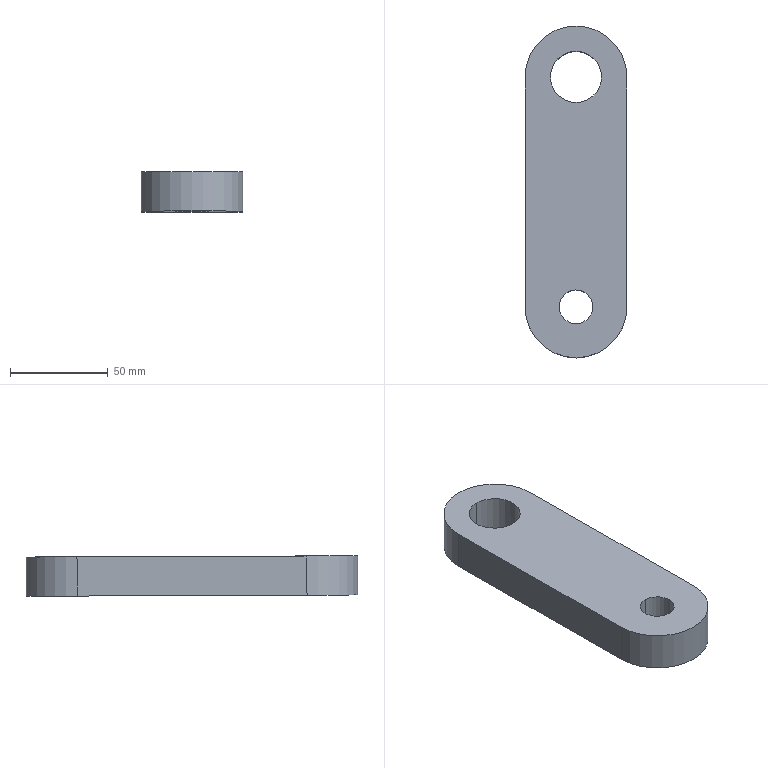Component | SolidWorks | RehabilitationChair-18-18-1 | 1 solid | 11 faces | box 52.03 x 169.45 x 20.64 mm | volume 149257 mm3 | cylinder 7 | plane 4 | commonest cylinder face diameters 52.026 x3 26.129 x2 17.187 x2
STEP:
#1=COLOUR_RGB('',0.7922,0.8196,0.9333);
#2=FILL_AREA_STYLE_COLOUR('',#1);
#3=FILL_AREA_STYLE('',(#2));
#4=SURFACE_STYLE_FILL_AREA(#3);
#5=SURFACE_SIDE_STYLE('',(#4));
#6=SURFACE_STYLE_USAGE(.BOTH.,#5);
#7=PRESENTATION_STYLE_ASSIGNMENT((#6));
#8=CARTESIAN_POINT('',(12.719,14.763,13.988));
#9=VERTEX_POINT('',#8);
#10=CARTESIAN_POINT('',(12.719,15.792,13.984));
#11=VERTEX_POINT('',#10);
#12=CARTESIAN_POINT('',(12.719,15.278,13.986));
#13=DIRECTION('',(-0.0003323,0.003798,1.));
#14=DIRECTION('',(0.,1.,-0.003798));
#15=AXIS2_PLACEMENT_3D('',#12,#13,#14);
#16=CIRCLE('',#15,0.5144);
#17=EDGE_CURVE('',#9,#11,#16,.T.);
#18=ORIENTED_EDGE('',*,*,#17,.T.);
#19=CARTESIAN_POINT('',(12.719,15.789,13.197));
#20=VERTEX_POINT('',#19);
#21=CARTESIAN_POINT('',(12.718,15.802,16.73));
#22=DIRECTION('',(0.0003323,-0.003798,-1.));
#23=VECTOR('',#22,39.37);
#24=LINE('',#21,#23);
#25=EDGE_CURVE('',#11,#20,#24,.T.);
#26=ORIENTED_EDGE('',*,*,#25,.T.);
#27=CARTESIAN_POINT('',(12.719,14.76,13.201));
#28=VERTEX_POINT('',#27);
#29=CARTESIAN_POINT('',(12.719,15.275,13.199));
#30=DIRECTION('',(-0.0003323,0.003798,1.));
#31=DIRECTION('',(0.,-1.,0.003798));
#32=AXIS2_PLACEMENT_3D('',#29,#30,#31);
#33=CIRCLE('',#32,0.5144);
#34=EDGE_CURVE('',#28,#20,#33,.T.);
#35=ORIENTED_EDGE('',*,*,#34,.F.);
#36=CARTESIAN_POINT('',(12.718,14.774,16.734));
#37=DIRECTION('',(0.0003323,-0.003798,-1.));
#38=VECTOR('',#37,39.37);
#39=LINE('',#36,#38);
#40=EDGE_CURVE('',#9,#28,#39,.T.);
#41=ORIENTED_EDGE('',*,*,#40,.F.);
#42=EDGE_LOOP('',(#18,#26,#35,#41));
#43=FACE_OUTER_BOUND('',#42,.T.);
#44=CARTESIAN_POINT('',(12.718,15.288,16.732));
#45=DIRECTION('',(0.0003323,-0.003798,-1.));
#46=DIRECTION('',(0.,-1.,0.003798));
#47=AXIS2_PLACEMENT_3D('',#44,#45,#46);
#48=CYLINDRICAL_SURFACE('',#47,0.5144);
#49=ADVANCED_FACE('',(#43),#48,.F.);
#50=CARTESIAN_POINT('',(12.719,10.996,14.002));
#51=VERTEX_POINT('',#50);
#52=CARTESIAN_POINT('',(12.719,10.319,14.005));
#53=VERTEX_POINT('',#52);
#54=CARTESIAN_POINT('',(12.719,10.658,14.004));
#55=DIRECTION('',(0.0003323,-0.003798,-1.));
#56=DIRECTION('',(0.,1.,-0.003798));
#57=AXIS2_PLACEMENT_3D('',#54,#55,#56);
#58=CIRCLE('',#57,0.3383);
#59=EDGE_CURVE('',#51,#53,#58,.T.);
#60=ORIENTED_EDGE('',*,*,#59,.F.);
#61=CARTESIAN_POINT('',(12.719,10.993,13.215));
#62=VERTEX_POINT('',#61);
#63=CARTESIAN_POINT('',(12.718,11.007,16.8));
#64=DIRECTION('',(0.0003323,-0.003798,-1.));
#65=VECTOR('',#64,39.37);
#66=LINE('',#63,#65);
#67=EDGE_CURVE('',#51,#62,#66,.T.);
#68=ORIENTED_EDGE('',*,*,#67,.T.);
#69=CARTESIAN_POINT('',(12.719,10.316,13.218));
#70=VERTEX_POINT('',#69);
#71=CARTESIAN_POINT('',(12.719,10.655,13.216));
#72=DIRECTION('',(-0.0003323,0.003798,1.));
#73=DIRECTION('',(0.,1.,-0.003798));
#74=AXIS2_PLACEMENT_3D('',#71,#72,#73);
#75=CIRCLE('',#74,0.3383);
#76=EDGE_CURVE('',#70,#62,#75,.T.);
#77=ORIENTED_EDGE('',*,*,#76,.F.);
#78=CARTESIAN_POINT('',(12.718,10.33,16.803));
#79=DIRECTION('',(0.0003323,-0.003798,-1.));
#80=VECTOR('',#79,39.37);
#81=LINE('',#78,#80);
#82=EDGE_CURVE('',#53,#70,#81,.T.);
#83=ORIENTED_EDGE('',*,*,#82,.F.);
#84=EDGE_LOOP('',(#60,#68,#77,#83));
#85=FACE_OUTER_BOUND('',#84,.T.);
#86=CARTESIAN_POINT('',(12.718,10.668,16.801));
#87=DIRECTION('',(0.0003323,-0.003798,-1.));
#88=DIRECTION('',(0.,-1.,0.003798));
#89=AXIS2_PLACEMENT_3D('',#86,#87,#88);
#90=CYLINDRICAL_SURFACE('',#89,0.3383);
#91=ADVANCED_FACE('',(#85),#90,.F.);
#92=CARTESIAN_POINT('',(13.743,15.275,13.199));
#93=VERTEX_POINT('',#92);
#94=CARTESIAN_POINT('',(12.719,16.299,13.195));
#95=VERTEX_POINT('',#94);
#96=CARTESIAN_POINT('',(12.719,15.275,13.199));
#97=DIRECTION('',(-0.0003323,0.003798,1.));
#98=DIRECTION('',(0.,-1.,0.003798));
#99=AXIS2_PLACEMENT_3D('',#96,#97,#98);
#100=CIRCLE('',#99,1.024);
#101=EDGE_CURVE('',#93,#95,#100,.T.);
#102=ORIENTED_EDGE('',*,*,#101,.T.);
#103=CARTESIAN_POINT('',(12.719,16.302,13.982));
#104=VERTEX_POINT('',#103);
#105=CARTESIAN_POINT('',(12.719,16.299,13.195));
#106=DIRECTION('',(-0.0003323,0.003798,1.));
#107=VECTOR('',#106,39.37);
#108=LINE('',#105,#107);
#109=EDGE_CURVE('',#95,#104,#108,.T.);
#110=ORIENTED_EDGE('',*,*,#109,.T.);
#111=CARTESIAN_POINT('',(13.743,15.278,13.986));
#112=VERTEX_POINT('',#111);
#113=CARTESIAN_POINT('',(12.719,15.278,13.986));
#114=DIRECTION('',(0.0003323,-0.003798,-1.));
#115=DIRECTION('',(0.,1.,-0.003798));
#116=AXIS2_PLACEMENT_3D('',#113,#114,#115);
#117=CIRCLE('',#116,1.024);
#118=EDGE_CURVE('',#104,#112,#117,.T.);
#119=ORIENTED_EDGE('',*,*,#118,.T.);
#120=CARTESIAN_POINT('',(13.743,15.275,13.199));
#121=DIRECTION('',(-0.0003323,0.003798,1.));
#122=VECTOR('',#121,39.37);
#123=LINE('',#120,#122);
#124=EDGE_CURVE('',#93,#112,#123,.T.);
#125=ORIENTED_EDGE('',*,*,#124,.F.);
#126=EDGE_LOOP('',(#102,#110,#119,#125));
#127=FACE_OUTER_BOUND('',#126,.T.);
#128=CARTESIAN_POINT('',(12.719,15.275,13.199));
#129=DIRECTION('',(-0.0003323,0.003798,1.));
#130=DIRECTION('',(0.,1.,-0.003798));
#131=AXIS2_PLACEMENT_3D('',#128,#129,#130);
#132=CYLINDRICAL_SURFACE('',#131,1.024);
#133=ADVANCED_FACE('',(#127),#132,.T.);
#134=ORIENTED_EDGE('',*,*,#109,.F.);
#135=CARTESIAN_POINT('',(11.695,15.275,13.198));
#136=VERTEX_POINT('',#135);
#137=CARTESIAN_POINT('',(12.719,15.275,13.199));
#138=DIRECTION('',(-0.0003323,0.003798,1.));
#139=DIRECTION('',(0.,-1.,0.003798));
#140=AXIS2_PLACEMENT_3D('',#137,#138,#139);
#141=CIRCLE('',#140,1.024);
#142=EDGE_CURVE('',#95,#136,#141,.T.);
#143=ORIENTED_EDGE('',*,*,#142,.T.);
#144=CARTESIAN_POINT('',(11.695,15.278,13.986));
#145=VERTEX_POINT('',#144);
#146=CARTESIAN_POINT('',(11.695,15.275,13.198));
#147=DIRECTION('',(-0.0003323,0.003798,1.));
#148=VECTOR('',#147,39.37);
#149=LINE('',#146,#148);
#150=EDGE_CURVE('',#136,#145,#149,.T.);
#151=ORIENTED_EDGE('',*,*,#150,.T.);
#152=CARTESIAN_POINT('',(12.719,15.278,13.986));
#153=DIRECTION('',(0.0003323,-0.003798,-1.));
#154=DIRECTION('',(0.,1.,-0.003798));
#155=AXIS2_PLACEMENT_3D('',#152,#153,#154);
#156=CIRCLE('',#155,1.024);
#157=EDGE_CURVE('',#145,#104,#156,.T.);
#158=ORIENTED_EDGE('',*,*,#157,.T.);
#159=EDGE_LOOP('',(#134,#143,#151,#158));
#160=FACE_OUTER_BOUND('',#159,.T.);
#161=CARTESIAN_POINT('',(12.719,15.275,13.199));
#162=DIRECTION('',(-0.0003323,0.003798,1.));
#163=DIRECTION('',(0.,1.,-0.003798));
#164=AXIS2_PLACEMENT_3D('',#161,#162,#163);
#165=CYLINDRICAL_SURFACE('',#164,1.024);
#166=ADVANCED_FACE('',(#160),#165,.T.);
#167=CARTESIAN_POINT('',(13.743,10.658,14.004));
#168=VERTEX_POINT('',#167);
#169=CARTESIAN_POINT('',(13.743,15.278,13.986));
#170=DIRECTION('',(0.,1.,-0.003798));
#171=VECTOR('',#170,39.37);
#172=LINE('',#169,#171);
#173=EDGE_CURVE('',#168,#112,#172,.T.);
#174=ORIENTED_EDGE('',*,*,#173,.F.);
#175=CARTESIAN_POINT('',(13.743,10.655,13.217));
#176=VERTEX_POINT('',#175);
#177=CARTESIAN_POINT('',(13.743,10.655,13.217));
#178=DIRECTION('',(-0.0003323,0.003798,1.));
#179=VECTOR('',#178,39.37);
#180=LINE('',#177,#179);
#181=EDGE_CURVE('',#176,#168,#180,.T.);
#182=ORIENTED_EDGE('',*,*,#181,.F.);
#183=CARTESIAN_POINT('',(13.743,15.275,13.199));
#184=DIRECTION('',(0.,1.,-0.003798));
#185=VECTOR('',#184,39.37);
#186=LINE('',#183,#185);
#187=EDGE_CURVE('',#176,#93,#186,.T.);
#188=ORIENTED_EDGE('',*,*,#187,.T.);
#189=ORIENTED_EDGE('',*,*,#124,.T.);
#190=EDGE_LOOP('',(#174,#182,#188,#189));
#191=FACE_OUTER_BOUND('',#190,.T.);
#192=CARTESIAN_POINT('',(13.743,15.275,13.199));
#193=DIRECTION('',(-1.,-0.00000126,-0.0003323));
#194=DIRECTION('',(0.0003323,0.,-1.));
#195=AXIS2_PLACEMENT_3D('',#192,#193,#194);
#196=PLANE('',#195);
#197=ADVANCED_FACE('',(#191),#196,.F.);
#198=CARTESIAN_POINT('',(11.695,10.658,14.003));
#199=VERTEX_POINT('',#198);
#200=CARTESIAN_POINT('',(11.695,15.278,13.986));
#201=DIRECTION('',(0.,-1.,0.003798));
#202=VECTOR('',#201,39.37);
#203=LINE('',#200,#202);
#204=EDGE_CURVE('',#145,#199,#203,.T.);
#205=ORIENTED_EDGE('',*,*,#204,.F.);
#206=ORIENTED_EDGE('',*,*,#150,.F.);
#207=CARTESIAN_POINT('',(11.695,10.655,13.216));
#208=VERTEX_POINT('',#207);
#209=CARTESIAN_POINT('',(11.695,15.275,13.198));
#210=DIRECTION('',(0.,-1.,0.003798));
#211=VECTOR('',#210,39.37);
#212=LINE('',#209,#211);
#213=EDGE_CURVE('',#136,#208,#212,.T.);
#214=ORIENTED_EDGE('',*,*,#213,.T.);
#215=CARTESIAN_POINT('',(11.695,10.655,13.216));
#216=DIRECTION('',(-0.0003323,0.003798,1.));
#217=VECTOR('',#216,39.37);
#218=LINE('',#215,#217);
#219=EDGE_CURVE('',#208,#199,#218,.T.);
#220=ORIENTED_EDGE('',*,*,#219,.T.);
#221=EDGE_LOOP('',(#205,#206,#214,#220));
#222=FACE_OUTER_BOUND('',#221,.T.);
#223=CARTESIAN_POINT('',(11.695,15.275,13.198));
#224=DIRECTION('',(1.,0.00000126,0.0003323));
#225=DIRECTION('',(-0.0003323,0.,1.));
#226=AXIS2_PLACEMENT_3D('',#223,#224,#225);
#227=PLANE('',#226);
#228=ADVANCED_FACE('',(#222),#227,.F.);
#229=CARTESIAN_POINT('',(12.719,10.658,14.004));
#230=DIRECTION('',(0.0003323,-0.003798,-1.));
#231=DIRECTION('',(0.,1.,-0.003798));
#232=AXIS2_PLACEMENT_3D('',#229,#230,#231);
#233=CIRCLE('',#232,0.3383);
#234=EDGE_CURVE('',#53,#51,#233,.T.);
#235=ORIENTED_EDGE('',*,*,#234,.T.);
#236=ORIENTED_EDGE('',*,*,#59,.T.);
#237=EDGE_LOOP('',(#235,#236));
#238=FACE_BOUND('',#237,.T.);
#239=ORIENTED_EDGE('',*,*,#17,.F.);
#240=CARTESIAN_POINT('',(12.719,15.278,13.986));
#241=DIRECTION('',(-0.0003323,0.003798,1.));
#242=DIRECTION('',(0.,1.,-0.003798));
#243=AXIS2_PLACEMENT_3D('',#240,#241,#242);
#244=CIRCLE('',#243,0.5144);
#245=EDGE_CURVE('',#11,#9,#244,.T.);
#246=ORIENTED_EDGE('',*,*,#245,.F.);
#247=EDGE_LOOP('',(#239,#246));
#248=FACE_BOUND('',#247,.T.);
#249=ORIENTED_EDGE('',*,*,#157,.F.);
#250=ORIENTED_EDGE('',*,*,#204,.T.);
#251=CARTESIAN_POINT('',(12.719,10.658,14.004));
#252=DIRECTION('',(-0.0003323,0.003798,1.));
#253=DIRECTION('',(0.,-1.,0.003798));
#254=AXIS2_PLACEMENT_3D('',#251,#252,#253);
#255=CIRCLE('',#254,1.024);
#256=EDGE_CURVE('',#199,#168,#255,.T.);
#257=ORIENTED_EDGE('',*,*,#256,.T.);
#258=ORIENTED_EDGE('',*,*,#173,.T.);
#259=ORIENTED_EDGE('',*,*,#118,.F.);
#260=EDGE_LOOP('',(#249,#250,#257,#258,#259));
#261=FACE_OUTER_BOUND('',#260,.T.);
#262=CARTESIAN_POINT('',(13.743,15.278,13.986));
#263=DIRECTION('',(-0.0003323,0.003798,1.));
#264=DIRECTION('',(0.,1.,-0.003798));
#265=AXIS2_PLACEMENT_3D('',#262,#263,#264);
#266=PLANE('',#265);
#267=ADVANCED_FACE('',(#238,#248,#261),#266,.T.);
#268=ORIENTED_EDGE('',*,*,#256,.F.);
#269=ORIENTED_EDGE('',*,*,#219,.F.);
#270=CARTESIAN_POINT('',(12.719,10.655,13.216));
#271=DIRECTION('',(-0.0003323,0.003798,1.));
#272=DIRECTION('',(0.,-1.,0.003798));
#273=AXIS2_PLACEMENT_3D('',#270,#271,#272);
#274=CIRCLE('',#273,1.024);
#275=EDGE_CURVE('',#208,#176,#274,.T.);
#276=ORIENTED_EDGE('',*,*,#275,.T.);
#277=ORIENTED_EDGE('',*,*,#181,.T.);
#278=EDGE_LOOP('',(#268,#269,#276,#277));
#279=FACE_OUTER_BOUND('',#278,.T.);
#280=CARTESIAN_POINT('',(12.719,10.655,13.216));
#281=DIRECTION('',(-0.0003323,0.003798,1.));
#282=DIRECTION('',(0.,1.,-0.003798));
#283=AXIS2_PLACEMENT_3D('',#280,#281,#282);
#284=CYLINDRICAL_SURFACE('',#283,1.024);
#285=ADVANCED_FACE('',(#279),#284,.T.);
#286=ORIENTED_EDGE('',*,*,#67,.F.);
#287=ORIENTED_EDGE('',*,*,#234,.F.);
#288=ORIENTED_EDGE('',*,*,#82,.T.);
#289=CARTESIAN_POINT('',(12.719,10.655,13.216));
#290=DIRECTION('',(-0.0003323,0.003798,1.));
#291=DIRECTION('',(0.,1.,-0.003798));
#292=AXIS2_PLACEMENT_3D('',#289,#290,#291);
#293=CIRCLE('',#292,0.3383);
#294=EDGE_CURVE('',#62,#70,#293,.T.);
#295=ORIENTED_EDGE('',*,*,#294,.F.);
#296=EDGE_LOOP('',(#286,#287,#288,#295));
#297=FACE_OUTER_BOUND('',#296,.T.);
#298=CARTESIAN_POINT('',(12.718,10.668,16.801));
#299=DIRECTION('',(0.0003323,-0.003798,-1.));
#300=DIRECTION('',(0.,-1.,0.003798));
#301=AXIS2_PLACEMENT_3D('',#298,#299,#300);
#302=CYLINDRICAL_SURFACE('',#301,0.3383);
#303=ADVANCED_FACE('',(#297),#302,.F.);
#304=ORIENTED_EDGE('',*,*,#25,.F.);
#305=ORIENTED_EDGE('',*,*,#245,.T.);
#306=ORIENTED_EDGE('',*,*,#40,.T.);
#307=CARTESIAN_POINT('',(12.719,15.275,13.199));
#308=DIRECTION('',(-0.0003323,0.003798,1.));
#309=DIRECTION('',(0.,-1.,0.003798));
#310=AXIS2_PLACEMENT_3D('',#307,#308,#309);
#311=CIRCLE('',#310,0.5144);
#312=EDGE_CURVE('',#20,#28,#311,.T.);
#313=ORIENTED_EDGE('',*,*,#312,.F.);
#314=EDGE_LOOP('',(#304,#305,#306,#313));
#315=FACE_OUTER_BOUND('',#314,.T.);
#316=CARTESIAN_POINT('',(12.718,15.288,16.732));
#317=DIRECTION('',(0.0003323,-0.003798,-1.));
#318=DIRECTION('',(0.,-1.,0.003798));
#319=AXIS2_PLACEMENT_3D('',#316,#317,#318);
#320=CYLINDRICAL_SURFACE('',#319,0.5144);
#321=ADVANCED_FACE('',(#315),#320,.F.);
#322=ORIENTED_EDGE('',*,*,#76,.T.);
#323=ORIENTED_EDGE('',*,*,#294,.T.);
#324=EDGE_LOOP('',(#322,#323));
#325=FACE_BOUND('',#324,.T.);
#326=ORIENTED_EDGE('',*,*,#275,.F.);
#327=ORIENTED_EDGE('',*,*,#213,.F.);
#328=ORIENTED_EDGE('',*,*,#142,.F.);
#329=ORIENTED_EDGE('',*,*,#101,.F.);
#330=ORIENTED_EDGE('',*,*,#187,.F.);
#331=EDGE_LOOP('',(#326,#327,#328,#329,#330));
#332=FACE_OUTER_BOUND('',#331,.T.);
#333=ORIENTED_EDGE('',*,*,#34,.T.);
#334=ORIENTED_EDGE('',*,*,#312,.T.);
#335=EDGE_LOOP('',(#333,#334));
#336=FACE_BOUND('',#335,.T.);
#337=CARTESIAN_POINT('',(13.39,11.335,13.214));
#338=DIRECTION('',(0.0003323,-0.003798,-1.));
#339=DIRECTION('',(0.,1.,-0.003798));
#340=AXIS2_PLACEMENT_3D('',#337,#338,#339);
#341=PLANE('',#340);
#342=ADVANCED_FACE('',(#325,#332,#336),#341,.T.);
#343=CLOSED_SHELL('',(#49,#91,#133,#166,#197,#228,#267,#285,#303,#321,#342));
#344=MANIFOLD_SOLID_BREP('',#343);
#345=STYLED_ITEM('',(#7),#344);
#346=PRESENTATION_LAYER_ASSIGNMENT('','',(#345));
#347=(LENGTH_UNIT()NAMED_UNIT(*)SI_UNIT($,.METRE.));
#348=LENGTH_MEASURE_WITH_UNIT(LENGTH_MEASURE(0.0254),#347);
#349=DIMENSIONAL_EXPONENTS(1.,0.,0.,0.,0.,0.,0.);
#350=(CONVERSION_BASED_UNIT('',#348)LENGTH_UNIT()NAMED_UNIT(#349));
#351=UNCERTAINTY_MEASURE_WITH_UNIT(LENGTH_MEASURE(0.00001),#350,'','');
#352=(NAMED_UNIT(*)PLANE_ANGLE_UNIT()SI_UNIT($,.RADIAN.));
#353=(NAMED_UNIT(*)SI_UNIT($,.STERADIAN.)SOLID_ANGLE_UNIT());
#354=(GEOMETRIC_REPRESENTATION_CONTEXT(3)GLOBAL_UNCERTAINTY_ASSIGNED_CONTEXT((#351))GLOBAL_UNIT_ASSIGNED_CONTEXT((#350,#352,#353))REPRESENTATION_CONTEXT('',''));
#355=MECHANICAL_DESIGN_GEOMETRIC_PRESENTATION_REPRESENTATION('',(#345),#354);
#356=CARTESIAN_POINT('',(0.,0.,0.));
#357=DIRECTION('',(0.,0.,1.));
#358=DIRECTION('',(1.,0.,0.));
#359=AXIS2_PLACEMENT_3D('',#356,#357,#358);
#360=(LENGTH_UNIT()NAMED_UNIT(*)SI_UNIT($,.METRE.));
#361=LENGTH_MEASURE_WITH_UNIT(LENGTH_MEASURE(0.0254),#360);
#362=DIMENSIONAL_EXPONENTS(1.,0.,0.,0.,0.,0.,0.);
#363=(CONVERSION_BASED_UNIT('',#361)LENGTH_UNIT()NAMED_UNIT(#362));
#364=UNCERTAINTY_MEASURE_WITH_UNIT(LENGTH_MEASURE(0.00001),#363,'','');
#365=(NAMED_UNIT(*)PLANE_ANGLE_UNIT()SI_UNIT($,.RADIAN.));
#366=(NAMED_UNIT(*)SI_UNIT($,.STERADIAN.)SOLID_ANGLE_UNIT());
#367=(GEOMETRIC_REPRESENTATION_CONTEXT(3)GLOBAL_UNCERTAINTY_ASSIGNED_CONTEXT((#364))GLOBAL_UNIT_ASSIGNED_CONTEXT((#363,#365,#366))REPRESENTATION_CONTEXT('',''));
#368=ADVANCED_BREP_SHAPE_REPRESENTATION('',(#344,#359),#367);